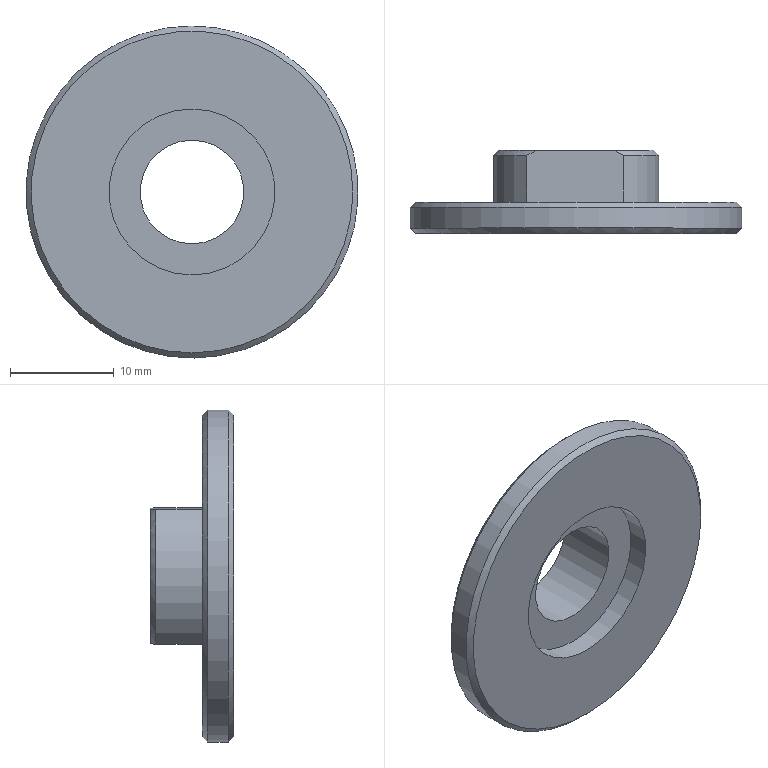Component | NX | LOCK_NUT | 1 solid | 15 faces | box 32 x 8 x 32 mm | volume 2421 mm3 | plane 6 | cylinder 5 | cone 4 | commonest cylinder face diameters 16 x3 32 x1 10 x1
STEP:
#1=CARTESIAN_POINT('',(0.,0.,0.));
#2=DIRECTION('',(0.,0.,1.));
#3=DIRECTION('',(1.,0.,0.));
#4=AXIS2_PLACEMENT_3D('',#1,#2,#3);
#5=CARTESIAN_POINT('',(-431.74,16.4,383.556));
#6=VERTEX_POINT('',#5);
#7=CARTESIAN_POINT('',(-431.676,16.4,378.556));
#8=DIRECTION('',(0.,-1.,0.));
#9=DIRECTION('',(-0.01278,0.,0.9999));
#10=AXIS2_PLACEMENT_3D('',#7,#8,#9);
#11=CIRCLE('',#10,5.);
#12=CARTESIAN_POINT('',(-423.676,16.4,378.658));
#13=DIRECTION('',(0.,-1.,0.));
#14=DIRECTION('',(-0.01278,0.,0.9999));
#15=AXIS2_PLACEMENT_3D('',#12,#13,#14);
#16=PLANE('',#15);
#17=CARTESIAN_POINT('',(-0.,8.));
#18=DIRECTION('',(1.,0.));
#19=AXIS2_PLACEMENT_2D('',#17,#18);
#20=CIRCLE('',#19,5.);
#21=(GEOMETRIC_REPRESENTATION_CONTEXT(2)PARAMETRIC_REPRESENTATION_CONTEXT()REPRESENTATION_CONTEXT('',''));
#22=DEFINITIONAL_REPRESENTATION('',(#20),#21);
#23=PCURVE('',#16,#22);
#24=CARTESIAN_POINT('',(-431.676,16.4,378.556));
#25=DIRECTION('',(0.,-1.,0.));
#26=DIRECTION('',(-0.01278,0.,0.9999));
#27=AXIS2_PLACEMENT_3D('',#24,#25,#26);
#28=CYLINDRICAL_SURFACE('',#27,5.);
#29=CARTESIAN_POINT('',(0.,0.));
#30=DIRECTION('',(1.,0.));
#31=VECTOR('',#30,1.);
#32=LINE('',#29,#31);
#33=(GEOMETRIC_REPRESENTATION_CONTEXT(2)PARAMETRIC_REPRESENTATION_CONTEXT()REPRESENTATION_CONTEXT('',''));
#34=DEFINITIONAL_REPRESENTATION('',(#32),#33);
#35=PCURVE('',#28,#34);
#36=SURFACE_CURVE('',#11,(#23,#35),.PCURVE_S1.);
#37=EDGE_CURVE('',#6,#6,#36,.T.);
#38=ORIENTED_EDGE('',*,*,#37,.T.);
#39=EDGE_LOOP('',(#38));
#40=FACE_BOUND('',#39,.T.);
#41=CARTESIAN_POINT('',(-428.017,16.4,385.103));
#42=VERTEX_POINT('',#41);
#43=CARTESIAN_POINT('',(-435.5,16.4,385.008));
#44=VERTEX_POINT('',#43);
#45=CARTESIAN_POINT('',(-423.759,16.4,385.158));
#46=DIRECTION('',(-0.9999,0.,-0.01278));
#47=VECTOR('',#46,1.);
#48=LINE('',#45,#47);
#49=CARTESIAN_POINT('',(6.5,-0.));
#50=DIRECTION('',(-0.,1.));
#51=VECTOR('',#50,1.);
#52=LINE('',#49,#51);
#53=(GEOMETRIC_REPRESENTATION_CONTEXT(2)PARAMETRIC_REPRESENTATION_CONTEXT()REPRESENTATION_CONTEXT('',''));
#54=DEFINITIONAL_REPRESENTATION('',(#52),#53);
#55=PCURVE('',#16,#54);
#56=CARTESIAN_POINT('',(-424.259,17.9,385.151));
#57=DIRECTION('',(-0.01278,0.,0.9999));
#58=DIRECTION('',(0.9999,0.,0.01278));
#59=AXIS2_PLACEMENT_3D('',#56,#57,#58);
#60=PLANE('',#59);
#61=CARTESIAN_POINT('',(0.5,-1.5));
#62=DIRECTION('',(-1.,0.));
#63=VECTOR('',#62,1.);
#64=LINE('',#61,#63);
#65=(GEOMETRIC_REPRESENTATION_CONTEXT(2)PARAMETRIC_REPRESENTATION_CONTEXT()REPRESENTATION_CONTEXT('',''));
#66=DEFINITIONAL_REPRESENTATION('',(#64),#65);
#67=PCURVE('',#60,#66);
#68=SURFACE_CURVE('',#48,(#55,#67),.PCURVE_S1.);
#69=EDGE_CURVE('',#42,#44,#68,.T.);
#70=ORIENTED_EDGE('',*,*,#69,.F.);
#71=CARTESIAN_POINT('',(-427.851,16.4,372.104));
#72=VERTEX_POINT('',#71);
#73=CARTESIAN_POINT('',(-431.676,16.4,378.556));
#74=DIRECTION('',(0.,1.,0.));
#75=DIRECTION('',(-0.01278,0.,0.9999));
#76=AXIS2_PLACEMENT_3D('',#73,#74,#75);
#77=CIRCLE('',#76,7.5);
#78=CARTESIAN_POINT('',(7.5,8.));
#79=CARTESIAN_POINT('',(7.5,-4.99));
#80=CARTESIAN_POINT('',(-3.75,1.505));
#81=CARTESIAN_POINT('',(-15.,8.));
#82=CARTESIAN_POINT('',(-3.75,14.495));
#83=CARTESIAN_POINT('',(7.5,20.99));
#84=CARTESIAN_POINT('',(7.5,8.));
#85=(BOUNDED_CURVE()B_SPLINE_CURVE(2,(#78,#79,#80,#81,#82,#83,#84),.UNSPECIFIED.,.T.,.F.)B_SPLINE_CURVE_WITH_KNOTS((1,2,2,2,2,1),(-2.094,0.,2.094,4.189,6.283,8.378),.UNSPECIFIED.)CURVE()GEOMETRIC_REPRESENTATION_ITEM()RATIONAL_B_SPLINE_CURVE((1.,0.5,1.,0.5,1.,0.5,1.))REPRESENTATION_ITEM(''));
#86=(GEOMETRIC_REPRESENTATION_CONTEXT(2)PARAMETRIC_REPRESENTATION_CONTEXT()REPRESENTATION_CONTEXT('',''));
#87=DEFINITIONAL_REPRESENTATION('',(#85),#86);
#88=PCURVE('',#16,#87);
#89=CARTESIAN_POINT('',(-431.676,16.4,378.556));
#90=DIRECTION('',(0.,-1.,0.));
#91=DIRECTION('',(-0.01278,0.,0.9999));
#92=AXIS2_PLACEMENT_3D('',#89,#90,#91);
#93=CONICAL_SURFACE('',#92,7.5,0.7854);
#94=CARTESIAN_POINT('',(6.283,-0.));
#95=DIRECTION('',(-1.,0.));
#96=VECTOR('',#95,1.);
#97=LINE('',#94,#96);
#98=(GEOMETRIC_REPRESENTATION_CONTEXT(2)PARAMETRIC_REPRESENTATION_CONTEXT()REPRESENTATION_CONTEXT('',''));
#99=DEFINITIONAL_REPRESENTATION('',(#97),#98);
#100=PCURVE('',#93,#99);
#101=SURFACE_CURVE('',#77,(#88,#100),.PCURVE_S1.);
#102=EDGE_CURVE('',#42,#72,#101,.T.);
#103=ORIENTED_EDGE('',*,*,#102,.T.);
#104=CARTESIAN_POINT('',(-435.334,16.4,372.009));
#105=VERTEX_POINT('',#104);
#106=CARTESIAN_POINT('',(-423.593,16.4,372.159));
#107=DIRECTION('',(0.9999,0.,0.01278));
#108=VECTOR('',#107,1.);
#109=LINE('',#106,#108);
#110=CARTESIAN_POINT('',(-6.5,0.));
#111=DIRECTION('',(-0.,-1.));
#112=VECTOR('',#111,1.);
#113=LINE('',#110,#112);
#114=(GEOMETRIC_REPRESENTATION_CONTEXT(2)PARAMETRIC_REPRESENTATION_CONTEXT()REPRESENTATION_CONTEXT('',''));
#115=DEFINITIONAL_REPRESENTATION('',(#113),#114);
#116=PCURVE('',#16,#115);
#117=CARTESIAN_POINT('',(-440.592,17.9,371.941));
#118=DIRECTION('',(0.01278,0.,-0.9999));
#119=DIRECTION('',(-0.9999,0.,-0.01278));
#120=AXIS2_PLACEMENT_3D('',#117,#118,#119);
#121=PLANE('',#120);
#122=CARTESIAN_POINT('',(-17.,-1.5));
#123=DIRECTION('',(-1.,0.));
#124=VECTOR('',#123,1.);
#125=LINE('',#122,#124);
#126=(GEOMETRIC_REPRESENTATION_CONTEXT(2)PARAMETRIC_REPRESENTATION_CONTEXT()REPRESENTATION_CONTEXT('',''));
#127=DEFINITIONAL_REPRESENTATION('',(#125),#126);
#128=PCURVE('',#121,#127);
#129=SURFACE_CURVE('',#109,(#116,#128),.PCURVE_S1.);
#130=EDGE_CURVE('',#105,#72,#129,.T.);
#131=ORIENTED_EDGE('',*,*,#130,.F.);
#132=CARTESIAN_POINT('',(-431.676,16.4,378.556));
#133=DIRECTION('',(0.,1.,0.));
#134=DIRECTION('',(-0.01278,0.,0.9999));
#135=AXIS2_PLACEMENT_3D('',#132,#133,#134);
#136=CIRCLE('',#135,7.5);
#137=CARTESIAN_POINT('',(7.5,8.));
#138=CARTESIAN_POINT('',(7.5,-4.99));
#139=CARTESIAN_POINT('',(-3.75,1.505));
#140=CARTESIAN_POINT('',(-15.,8.));
#141=CARTESIAN_POINT('',(-3.75,14.495));
#142=CARTESIAN_POINT('',(7.5,20.99));
#143=CARTESIAN_POINT('',(7.5,8.));
#144=(BOUNDED_CURVE()B_SPLINE_CURVE(2,(#137,#138,#139,#140,#141,#142,#143),.UNSPECIFIED.,.T.,.F.)B_SPLINE_CURVE_WITH_KNOTS((1,2,2,2,2,1),(-2.094,0.,2.094,4.189,6.283,8.378),.UNSPECIFIED.)CURVE()GEOMETRIC_REPRESENTATION_ITEM()RATIONAL_B_SPLINE_CURVE((1.,0.5,1.,0.5,1.,0.5,1.))REPRESENTATION_ITEM(''));
#145=(GEOMETRIC_REPRESENTATION_CONTEXT(2)PARAMETRIC_REPRESENTATION_CONTEXT()REPRESENTATION_CONTEXT('',''));
#146=DEFINITIONAL_REPRESENTATION('',(#144),#145);
#147=PCURVE('',#16,#146);
#148=CARTESIAN_POINT('',(-431.676,16.4,378.556));
#149=DIRECTION('',(0.,-1.,0.));
#150=DIRECTION('',(-0.01278,0.,0.9999));
#151=AXIS2_PLACEMENT_3D('',#148,#149,#150);
#152=CONICAL_SURFACE('',#151,7.5,0.7854);
#153=CARTESIAN_POINT('',(6.283,0.));
#154=DIRECTION('',(-1.,-0.));
#155=VECTOR('',#154,1.);
#156=LINE('',#153,#155);
#157=(GEOMETRIC_REPRESENTATION_CONTEXT(2)PARAMETRIC_REPRESENTATION_CONTEXT()REPRESENTATION_CONTEXT('',''));
#158=DEFINITIONAL_REPRESENTATION('',(#156),#157);
#159=PCURVE('',#152,#158);
#160=SURFACE_CURVE('',#136,(#147,#159),.PCURVE_S1.);
#161=EDGE_CURVE('',#105,#44,#160,.T.);
#162=ORIENTED_EDGE('',*,*,#161,.T.);
#163=EDGE_LOOP('',(#70,#103,#131,#162));
#164=FACE_BOUND('',#163,.T.);
#165=ADVANCED_FACE('',(#40,#164),#16,.F.);
#166=CARTESIAN_POINT('',(-426.929,15.9,372.116));
#167=VERTEX_POINT('',#166);
#168=CARTESIAN_POINT('',(-426.929,11.4,372.116));
#169=VERTEX_POINT('',#168);
#170=CARTESIAN_POINT('',(-426.929,8.4,372.116));
#171=DIRECTION('',(0.,-1.,0.));
#172=VECTOR('',#171,1.);
#173=LINE('',#170,#172);
#174=CARTESIAN_POINT('',(-431.676,8.4,378.556));
#175=DIRECTION('',(0.,1.,0.));
#176=DIRECTION('',(0.01278,0.,-0.9999));
#177=AXIS2_PLACEMENT_3D('',#174,#175,#176);
#178=CYLINDRICAL_SURFACE('',#177,8.);
#179=CARTESIAN_POINT('',(5.661,0.));
#180=DIRECTION('',(0.,-1.));
#181=VECTOR('',#180,1.);
#182=LINE('',#179,#181);
#183=(GEOMETRIC_REPRESENTATION_CONTEXT(2)PARAMETRIC_REPRESENTATION_CONTEXT()REPRESENTATION_CONTEXT('',''));
#184=DEFINITIONAL_REPRESENTATION('',(#182),#183);
#185=PCURVE('',#178,#184);
#186=CARTESIAN_POINT('',(-13.664,-9.5));
#187=DIRECTION('',(0.,-1.));
#188=VECTOR('',#187,1.);
#189=LINE('',#186,#188);
#190=(GEOMETRIC_REPRESENTATION_CONTEXT(2)PARAMETRIC_REPRESENTATION_CONTEXT()REPRESENTATION_CONTEXT('',''));
#191=DEFINITIONAL_REPRESENTATION('',(#189),#190);
#192=PCURVE('',#121,#191);
#193=SURFACE_CURVE('',#173,(#185,#192),.PCURVE_S1.);
#194=EDGE_CURVE('',#167,#169,#193,.T.);
#195=ORIENTED_EDGE('',*,*,#194,.F.);
#196=CARTESIAN_POINT('',(-427.095,15.9,385.115));
#197=VERTEX_POINT('',#196);
#198=CARTESIAN_POINT('',(-431.676,15.9,378.556));
#199=DIRECTION('',(0.,-1.,0.));
#200=DIRECTION('',(-0.01278,0.,0.9999));
#201=AXIS2_PLACEMENT_3D('',#198,#199,#200);
#202=CIRCLE('',#201,8.);
#203=CARTESIAN_POINT('',(9.425,7.5));
#204=DIRECTION('',(-1.,0.));
#205=VECTOR('',#204,1.);
#206=LINE('',#203,#205);
#207=(GEOMETRIC_REPRESENTATION_CONTEXT(2)PARAMETRIC_REPRESENTATION_CONTEXT()REPRESENTATION_CONTEXT('',''));
#208=DEFINITIONAL_REPRESENTATION('',(#206),#207);
#209=PCURVE('',#178,#208);
#210=CARTESIAN_POINT('',(-0.,0.5));
#211=DIRECTION('',(1.,-0.));
#212=VECTOR('',#211,1.);
#213=LINE('',#210,#212);
#214=(GEOMETRIC_REPRESENTATION_CONTEXT(2)PARAMETRIC_REPRESENTATION_CONTEXT()REPRESENTATION_CONTEXT('',''));
#215=DEFINITIONAL_REPRESENTATION('',(#213),#214);
#216=PCURVE('',#93,#215);
#217=SURFACE_CURVE('',#202,(#209,#216),.PCURVE_S1.);
#218=EDGE_CURVE('',#167,#197,#217,.T.);
#219=ORIENTED_EDGE('',*,*,#218,.T.);
#220=CARTESIAN_POINT('',(-427.095,11.4,385.115));
#221=VERTEX_POINT('',#220);
#222=CARTESIAN_POINT('',(-427.095,8.4,385.115));
#223=DIRECTION('',(0.,1.,0.));
#224=VECTOR('',#223,1.);
#225=LINE('',#222,#224);
#226=CARTESIAN_POINT('',(3.764,0.));
#227=DIRECTION('',(0.,1.));
#228=VECTOR('',#227,1.);
#229=LINE('',#226,#228);
#230=(GEOMETRIC_REPRESENTATION_CONTEXT(2)PARAMETRIC_REPRESENTATION_CONTEXT()REPRESENTATION_CONTEXT('',''));
#231=DEFINITIONAL_REPRESENTATION('',(#229),#230);
#232=PCURVE('',#178,#231);
#233=CARTESIAN_POINT('',(-2.836,-9.5));
#234=DIRECTION('',(0.,1.));
#235=VECTOR('',#234,1.);
#236=LINE('',#233,#235);
#237=(GEOMETRIC_REPRESENTATION_CONTEXT(2)PARAMETRIC_REPRESENTATION_CONTEXT()REPRESENTATION_CONTEXT('',''));
#238=DEFINITIONAL_REPRESENTATION('',(#236),#237);
#239=PCURVE('',#60,#238);
#240=SURFACE_CURVE('',#225,(#232,#239),.PCURVE_S1.);
#241=EDGE_CURVE('',#221,#197,#240,.T.);
#242=ORIENTED_EDGE('',*,*,#241,.F.);
#243=CARTESIAN_POINT('',(-431.676,11.4,378.556));
#244=DIRECTION('',(0.,1.,0.));
#245=DIRECTION('',(0.01278,0.,-0.9999));
#246=AXIS2_PLACEMENT_3D('',#243,#244,#245);
#247=CIRCLE('',#246,8.);
#248=CARTESIAN_POINT('',(0.,3.));
#249=DIRECTION('',(1.,0.));
#250=VECTOR('',#249,1.);
#251=LINE('',#248,#250);
#252=(GEOMETRIC_REPRESENTATION_CONTEXT(2)PARAMETRIC_REPRESENTATION_CONTEXT()REPRESENTATION_CONTEXT('',''));
#253=DEFINITIONAL_REPRESENTATION('',(#251),#252);
#254=PCURVE('',#178,#253);
#255=CARTESIAN_POINT('',(-415.677,11.4,378.76));
#256=DIRECTION('',(0.,-1.,0.));
#257=DIRECTION('',(-0.01278,0.,0.9999));
#258=AXIS2_PLACEMENT_3D('',#255,#256,#257);
#259=PLANE('',#258);
#260=CARTESIAN_POINT('',(-8.,16.));
#261=CARTESIAN_POINT('',(-8.,29.856));
#262=CARTESIAN_POINT('',(4.,22.928));
#263=CARTESIAN_POINT('',(16.,16.));
#264=CARTESIAN_POINT('',(4.,9.072));
#265=CARTESIAN_POINT('',(-8.,2.144));
#266=CARTESIAN_POINT('',(-8.,16.));
#267=(BOUNDED_CURVE()B_SPLINE_CURVE(2,(#260,#261,#262,#263,#264,#265,#266),.UNSPECIFIED.,.T.,.F.)B_SPLINE_CURVE_WITH_KNOTS((1,2,2,2,2,1),(-2.094,0.,2.094,4.189,6.283,8.378),.UNSPECIFIED.)CURVE()GEOMETRIC_REPRESENTATION_ITEM()RATIONAL_B_SPLINE_CURVE((1.,0.5,1.,0.5,1.,0.5,1.))REPRESENTATION_ITEM(''));
#268=(GEOMETRIC_REPRESENTATION_CONTEXT(2)PARAMETRIC_REPRESENTATION_CONTEXT()REPRESENTATION_CONTEXT('',''));
#269=DEFINITIONAL_REPRESENTATION('',(#267),#268);
#270=PCURVE('',#259,#269);
#271=SURFACE_CURVE('',#247,(#254,#270),.PCURVE_S1.);
#272=EDGE_CURVE('',#221,#169,#271,.T.);
#273=ORIENTED_EDGE('',*,*,#272,.T.);
#274=EDGE_LOOP('',(#195,#219,#242,#273));
#275=FACE_BOUND('',#274,.T.);
#276=ADVANCED_FACE('',(#275),#178,.T.);
#277=CARTESIAN_POINT('',(-436.422,15.9,384.996));
#278=VERTEX_POINT('',#277);
#279=CARTESIAN_POINT('',(-436.422,11.4,384.996));
#280=VERTEX_POINT('',#279);
#281=CARTESIAN_POINT('',(-436.422,8.4,384.996));
#282=DIRECTION('',(0.,-1.,0.));
#283=VECTOR('',#282,1.);
#284=LINE('',#281,#283);
#285=CARTESIAN_POINT('',(-431.676,8.4,378.556));
#286=DIRECTION('',(0.,1.,0.));
#287=DIRECTION('',(0.01278,0.,-0.9999));
#288=AXIS2_PLACEMENT_3D('',#285,#286,#287);
#289=CYLINDRICAL_SURFACE('',#288,8.);
#290=CARTESIAN_POINT('',(2.519,0.));
#291=DIRECTION('',(0.,-1.));
#292=VECTOR('',#291,1.);
#293=LINE('',#290,#292);
#294=(GEOMETRIC_REPRESENTATION_CONTEXT(2)PARAMETRIC_REPRESENTATION_CONTEXT()REPRESENTATION_CONTEXT('',''));
#295=DEFINITIONAL_REPRESENTATION('',(#293),#294);
#296=PCURVE('',#289,#295);
#297=CARTESIAN_POINT('',(-12.164,-9.5));
#298=DIRECTION('',(0.,-1.));
#299=VECTOR('',#298,1.);
#300=LINE('',#297,#299);
#301=(GEOMETRIC_REPRESENTATION_CONTEXT(2)PARAMETRIC_REPRESENTATION_CONTEXT()REPRESENTATION_CONTEXT('',''));
#302=DEFINITIONAL_REPRESENTATION('',(#300),#301);
#303=PCURVE('',#60,#302);
#304=SURFACE_CURVE('',#284,(#296,#303),.PCURVE_S1.);
#305=EDGE_CURVE('',#278,#280,#304,.T.);
#306=ORIENTED_EDGE('',*,*,#305,.F.);
#307=CARTESIAN_POINT('',(-436.256,15.9,371.997));
#308=VERTEX_POINT('',#307);
#309=CARTESIAN_POINT('',(-431.676,15.9,378.556));
#310=DIRECTION('',(0.,-1.,0.));
#311=DIRECTION('',(-0.01278,0.,0.9999));
#312=AXIS2_PLACEMENT_3D('',#309,#310,#311);
#313=CIRCLE('',#312,8.);
#314=CARTESIAN_POINT('',(3.142,7.5));
#315=DIRECTION('',(-1.,0.));
#316=VECTOR('',#315,1.);
#317=LINE('',#314,#316);
#318=(GEOMETRIC_REPRESENTATION_CONTEXT(2)PARAMETRIC_REPRESENTATION_CONTEXT()REPRESENTATION_CONTEXT('',''));
#319=DEFINITIONAL_REPRESENTATION('',(#317),#318);
#320=PCURVE('',#289,#319);
#321=CARTESIAN_POINT('',(-0.,0.5));
#322=DIRECTION('',(1.,0.));
#323=VECTOR('',#322,1.);
#324=LINE('',#321,#323);
#325=(GEOMETRIC_REPRESENTATION_CONTEXT(2)PARAMETRIC_REPRESENTATION_CONTEXT()REPRESENTATION_CONTEXT('',''));
#326=DEFINITIONAL_REPRESENTATION('',(#324),#325);
#327=PCURVE('',#152,#326);
#328=SURFACE_CURVE('',#313,(#320,#327),.PCURVE_S1.);
#329=EDGE_CURVE('',#278,#308,#328,.T.);
#330=ORIENTED_EDGE('',*,*,#329,.T.);
#331=CARTESIAN_POINT('',(-436.256,11.4,371.997));
#332=VERTEX_POINT('',#331);
#333=CARTESIAN_POINT('',(-436.256,8.4,371.997));
#334=DIRECTION('',(0.,1.,0.));
#335=VECTOR('',#334,1.);
#336=LINE('',#333,#335);
#337=CARTESIAN_POINT('',(0.6224,0.));
#338=DIRECTION('',(0.,1.));
#339=VECTOR('',#338,1.);
#340=LINE('',#337,#339);
#341=(GEOMETRIC_REPRESENTATION_CONTEXT(2)PARAMETRIC_REPRESENTATION_CONTEXT()REPRESENTATION_CONTEXT('',''));
#342=DEFINITIONAL_REPRESENTATION('',(#340),#341);
#343=PCURVE('',#289,#342);
#344=CARTESIAN_POINT('',(-4.336,-9.5));
#345=DIRECTION('',(0.,1.));
#346=VECTOR('',#345,1.);
#347=LINE('',#344,#346);
#348=(GEOMETRIC_REPRESENTATION_CONTEXT(2)PARAMETRIC_REPRESENTATION_CONTEXT()REPRESENTATION_CONTEXT('',''));
#349=DEFINITIONAL_REPRESENTATION('',(#347),#348);
#350=PCURVE('',#121,#349);
#351=SURFACE_CURVE('',#336,(#343,#350),.PCURVE_S1.);
#352=EDGE_CURVE('',#332,#308,#351,.T.);
#353=ORIENTED_EDGE('',*,*,#352,.F.);
#354=CARTESIAN_POINT('',(-431.676,11.4,378.556));
#355=DIRECTION('',(0.,1.,0.));
#356=DIRECTION('',(0.01278,0.,-0.9999));
#357=AXIS2_PLACEMENT_3D('',#354,#355,#356);
#358=CIRCLE('',#357,8.);
#359=CARTESIAN_POINT('',(-0.,3.));
#360=DIRECTION('',(1.,0.));
#361=VECTOR('',#360,1.);
#362=LINE('',#359,#361);
#363=(GEOMETRIC_REPRESENTATION_CONTEXT(2)PARAMETRIC_REPRESENTATION_CONTEXT()REPRESENTATION_CONTEXT('',''));
#364=DEFINITIONAL_REPRESENTATION('',(#362),#363);
#365=PCURVE('',#289,#364);
#366=CARTESIAN_POINT('',(-8.,16.));
#367=CARTESIAN_POINT('',(-8.,29.856));
#368=CARTESIAN_POINT('',(4.,22.928));
#369=CARTESIAN_POINT('',(16.,16.));
#370=CARTESIAN_POINT('',(4.,9.072));
#371=CARTESIAN_POINT('',(-8.,2.144));
#372=CARTESIAN_POINT('',(-8.,16.));
#373=(BOUNDED_CURVE()B_SPLINE_CURVE(2,(#366,#367,#368,#369,#370,#371,#372),.UNSPECIFIED.,.T.,.F.)B_SPLINE_CURVE_WITH_KNOTS((1,2,2,2,2,1),(-2.094,0.,2.094,4.189,6.283,8.378),.UNSPECIFIED.)CURVE()GEOMETRIC_REPRESENTATION_ITEM()RATIONAL_B_SPLINE_CURVE((1.,0.5,1.,0.5,1.,0.5,1.))REPRESENTATION_ITEM(''));
#374=(GEOMETRIC_REPRESENTATION_CONTEXT(2)PARAMETRIC_REPRESENTATION_CONTEXT()REPRESENTATION_CONTEXT('',''));
#375=DEFINITIONAL_REPRESENTATION('',(#373),#374);
#376=PCURVE('',#259,#375);
#377=SURFACE_CURVE('',#358,(#365,#376),.PCURVE_S1.);
#378=EDGE_CURVE('',#332,#280,#377,.T.);
#379=ORIENTED_EDGE('',*,*,#378,.T.);
#380=EDGE_LOOP('',(#306,#330,#353,#379));
#381=FACE_BOUND('',#380,.T.);
#382=ADVANCED_FACE('',(#381),#289,.T.);
#383=CARTESIAN_POINT('',(-431.874,11.4,394.055));
#384=VERTEX_POINT('',#383);
#385=CARTESIAN_POINT('',(-431.676,11.4,378.556));
#386=DIRECTION('',(0.,1.,0.));
#387=DIRECTION('',(-0.01278,0.,0.9999));
#388=AXIS2_PLACEMENT_3D('',#385,#386,#387);
#389=CIRCLE('',#388,15.5);
#390=CARTESIAN_POINT('',(15.5,16.));
#391=CARTESIAN_POINT('',(15.5,-10.847));
#392=CARTESIAN_POINT('',(-7.75,2.577));
#393=CARTESIAN_POINT('',(-31.,16.));
#394=CARTESIAN_POINT('',(-7.75,29.423));
#395=CARTESIAN_POINT('',(15.5,42.847));
#396=CARTESIAN_POINT('',(15.5,16.));
#397=(BOUNDED_CURVE()B_SPLINE_CURVE(2,(#390,#391,#392,#393,#394,#395,#396),.UNSPECIFIED.,.T.,.F.)B_SPLINE_CURVE_WITH_KNOTS((1,2,2,2,2,1),(-2.094,0.,2.094,4.189,6.283,8.378),.UNSPECIFIED.)CURVE()GEOMETRIC_REPRESENTATION_ITEM()RATIONAL_B_SPLINE_CURVE((1.,0.5,1.,0.5,1.,0.5,1.))REPRESENTATION_ITEM(''));
#398=(GEOMETRIC_REPRESENTATION_CONTEXT(2)PARAMETRIC_REPRESENTATION_CONTEXT()REPRESENTATION_CONTEXT('',''));
#399=DEFINITIONAL_REPRESENTATION('',(#397),#398);
#400=PCURVE('',#259,#399);
#401=CARTESIAN_POINT('',(-431.676,11.4,378.556));
#402=DIRECTION('',(0.,-1.,0.));
#403=DIRECTION('',(-0.01278,0.,0.9999));
#404=AXIS2_PLACEMENT_3D('',#401,#402,#403);
#405=CONICAL_SURFACE('',#404,15.5,0.7854);
#406=CARTESIAN_POINT('',(6.283,-0.));
#407=DIRECTION('',(-1.,0.));
#408=VECTOR('',#407,1.);
#409=LINE('',#406,#408);
#410=(GEOMETRIC_REPRESENTATION_CONTEXT(2)PARAMETRIC_REPRESENTATION_CONTEXT()REPRESENTATION_CONTEXT('',''));
#411=DEFINITIONAL_REPRESENTATION('',(#409),#410);
#412=PCURVE('',#405,#411);
#413=SURFACE_CURVE('',#389,(#400,#412),.PCURVE_S1.);
#414=EDGE_CURVE('',#384,#384,#413,.T.);
#415=ORIENTED_EDGE('',*,*,#414,.T.);
#416=EDGE_LOOP('',(#415));
#417=FACE_BOUND('',#416,.T.);
#418=ORIENTED_EDGE('',*,*,#272,.F.);
#419=CARTESIAN_POINT('',(-424.259,11.4,385.151));
#420=DIRECTION('',(-0.9999,0.,-0.01278));
#421=VECTOR('',#420,1.);
#422=LINE('',#419,#421);
#423=CARTESIAN_POINT('',(6.5,8.5));
#424=DIRECTION('',(-0.,1.));
#425=VECTOR('',#424,1.);
#426=LINE('',#423,#425);
#427=(GEOMETRIC_REPRESENTATION_CONTEXT(2)PARAMETRIC_REPRESENTATION_CONTEXT()REPRESENTATION_CONTEXT('',''));
#428=DEFINITIONAL_REPRESENTATION('',(#426),#427);
#429=PCURVE('',#259,#428);
#430=CARTESIAN_POINT('',(0.,-6.5));
#431=DIRECTION('',(-1.,0.));
#432=VECTOR('',#431,1.);
#433=LINE('',#430,#432);
#434=(GEOMETRIC_REPRESENTATION_CONTEXT(2)PARAMETRIC_REPRESENTATION_CONTEXT()REPRESENTATION_CONTEXT('',''));
#435=DEFINITIONAL_REPRESENTATION('',(#433),#434);
#436=PCURVE('',#60,#435);
#437=SURFACE_CURVE('',#422,(#429,#436),.PCURVE_S1.);
#438=EDGE_CURVE('',#221,#280,#437,.T.);
#439=ORIENTED_EDGE('',*,*,#438,.T.);
#440=ORIENTED_EDGE('',*,*,#378,.F.);
#441=CARTESIAN_POINT('',(-440.592,11.4,371.941));
#442=DIRECTION('',(0.9999,0.,0.01278));
#443=VECTOR('',#442,1.);
#444=LINE('',#441,#443);
#445=CARTESIAN_POINT('',(-6.5,25.));
#446=DIRECTION('',(-0.,-1.));
#447=VECTOR('',#446,1.);
#448=LINE('',#445,#447);
#449=(GEOMETRIC_REPRESENTATION_CONTEXT(2)PARAMETRIC_REPRESENTATION_CONTEXT()REPRESENTATION_CONTEXT('',''));
#450=DEFINITIONAL_REPRESENTATION('',(#448),#449);
#451=PCURVE('',#259,#450);
#452=CARTESIAN_POINT('',(0.,-6.5));
#453=DIRECTION('',(-1.,0.));
#454=VECTOR('',#453,1.);
#455=LINE('',#452,#454);
#456=(GEOMETRIC_REPRESENTATION_CONTEXT(2)PARAMETRIC_REPRESENTATION_CONTEXT()REPRESENTATION_CONTEXT('',''));
#457=DEFINITIONAL_REPRESENTATION('',(#455),#456);
#458=PCURVE('',#121,#457);
#459=SURFACE_CURVE('',#444,(#451,#458),.PCURVE_S1.);
#460=EDGE_CURVE('',#332,#169,#459,.T.);
#461=ORIENTED_EDGE('',*,*,#460,.T.);
#462=EDGE_LOOP('',(#418,#439,#440,#461));
#463=FACE_BOUND('',#462,.T.);
#464=ADVANCED_FACE('',(#417,#463),#259,.F.);
#465=CARTESIAN_POINT('',(-431.471,8.9,362.557));
#466=VERTEX_POINT('',#465);
#467=CARTESIAN_POINT('',(-431.676,8.9,378.556));
#468=DIRECTION('',(0.,1.,0.));
#469=DIRECTION('',(0.01278,0.,-0.9999));
#470=AXIS2_PLACEMENT_3D('',#467,#468,#469);
#471=CIRCLE('',#470,16.);
#472=CARTESIAN_POINT('',(-431.676,8.4,378.556));
#473=DIRECTION('',(0.,1.,0.));
#474=DIRECTION('',(0.01278,0.,-0.9999));
#475=AXIS2_PLACEMENT_3D('',#472,#473,#474);
#476=CYLINDRICAL_SURFACE('',#475,16.);
#477=CARTESIAN_POINT('',(0.,0.5));
#478=DIRECTION('',(1.,0.));
#479=VECTOR('',#478,1.);
#480=LINE('',#477,#479);
#481=(GEOMETRIC_REPRESENTATION_CONTEXT(2)PARAMETRIC_REPRESENTATION_CONTEXT()REPRESENTATION_CONTEXT('',''));
#482=DEFINITIONAL_REPRESENTATION('',(#480),#481);
#483=PCURVE('',#476,#482);
#484=CARTESIAN_POINT('',(-431.676,8.9,378.556));
#485=DIRECTION('',(0.,1.,0.));
#486=DIRECTION('',(0.01278,0.,-0.9999));
#487=AXIS2_PLACEMENT_3D('',#484,#485,#486);
#488=CONICAL_SURFACE('',#487,16.,0.7854);
#489=CARTESIAN_POINT('',(0.,0.));
#490=DIRECTION('',(1.,0.));
#491=VECTOR('',#490,1.);
#492=LINE('',#489,#491);
#493=(GEOMETRIC_REPRESENTATION_CONTEXT(2)PARAMETRIC_REPRESENTATION_CONTEXT()REPRESENTATION_CONTEXT('',''));
#494=DEFINITIONAL_REPRESENTATION('',(#492),#493);
#495=PCURVE('',#488,#494);
#496=SURFACE_CURVE('',#471,(#483,#495),.PCURVE_S1.);
#497=EDGE_CURVE('',#466,#466,#496,.T.);
#498=ORIENTED_EDGE('',*,*,#497,.T.);
#499=CARTESIAN_POINT('',(-431.471,10.9,362.557));
#500=VERTEX_POINT('',#499);
#501=CARTESIAN_POINT('',(-431.471,8.9,362.557));
#502=CARTESIAN_POINT('',(-431.471,10.9,362.557));
#503=B_SPLINE_CURVE_WITH_KNOTS('',1,(#501,#502),.UNSPECIFIED.,.F.,.F.,(2,2),(0.5,2.5),.PIECEWISE_BEZIER_KNOTS.);
#504=CARTESIAN_POINT('',(6.283,0.));
#505=DIRECTION('',(0.,1.));
#506=VECTOR('',#505,1.);
#507=LINE('',#504,#506);
#508=(GEOMETRIC_REPRESENTATION_CONTEXT(2)PARAMETRIC_REPRESENTATION_CONTEXT()REPRESENTATION_CONTEXT('',''));
#509=DEFINITIONAL_REPRESENTATION('',(#507),#508);
#510=PCURVE('',#476,#509);
#511=CARTESIAN_POINT('',(0.,0.));
#512=DIRECTION('',(0.,1.));
#513=VECTOR('',#512,1.);
#514=LINE('',#511,#513);
#515=(GEOMETRIC_REPRESENTATION_CONTEXT(2)PARAMETRIC_REPRESENTATION_CONTEXT()REPRESENTATION_CONTEXT('',''));
#516=DEFINITIONAL_REPRESENTATION('',(#514),#515);
#517=PCURVE('',#476,#516);
#518=SEAM_CURVE('',#503,(#510,#517),.PCURVE_S1.);
#519=EDGE_CURVE('',#466,#500,#518,.T.);
#520=ORIENTED_EDGE('',*,*,#519,.T.);
#521=CARTESIAN_POINT('',(-431.88,10.9,394.555));
#522=VERTEX_POINT('',#521);
#523=CARTESIAN_POINT('',(-431.676,10.9,378.556));
#524=DIRECTION('',(0.,-1.,0.));
#525=DIRECTION('',(-0.01278,0.,0.9999));
#526=AXIS2_PLACEMENT_3D('',#523,#524,#525);
#527=CIRCLE('',#526,16.);
#528=CARTESIAN_POINT('',(9.425,2.5));
#529=DIRECTION('',(-1.,0.));
#530=VECTOR('',#529,1.);
#531=LINE('',#528,#530);
#532=(GEOMETRIC_REPRESENTATION_CONTEXT(2)PARAMETRIC_REPRESENTATION_CONTEXT()REPRESENTATION_CONTEXT('',''));
#533=DEFINITIONAL_REPRESENTATION('',(#531),#532);
#534=PCURVE('',#476,#533);
#535=CARTESIAN_POINT('',(0.,0.5));
#536=DIRECTION('',(1.,-0.));
#537=VECTOR('',#536,1.);
#538=LINE('',#535,#537);
#539=(GEOMETRIC_REPRESENTATION_CONTEXT(2)PARAMETRIC_REPRESENTATION_CONTEXT()REPRESENTATION_CONTEXT('',''));
#540=DEFINITIONAL_REPRESENTATION('',(#538),#539);
#541=PCURVE('',#405,#540);
#542=SURFACE_CURVE('',#527,(#534,#541),.PCURVE_S1.);
#543=EDGE_CURVE('',#500,#522,#542,.T.);
#544=ORIENTED_EDGE('',*,*,#543,.T.);
#545=CARTESIAN_POINT('',(-431.676,10.9,378.556));
#546=DIRECTION('',(0.,-1.,0.));
#547=DIRECTION('',(-0.01278,0.,0.9999));
#548=AXIS2_PLACEMENT_3D('',#545,#546,#547);
#549=CIRCLE('',#548,16.);
#550=CARTESIAN_POINT('',(3.142,2.5));
#551=DIRECTION('',(-1.,0.));
#552=VECTOR('',#551,1.);
#553=LINE('',#550,#552);
#554=(GEOMETRIC_REPRESENTATION_CONTEXT(2)PARAMETRIC_REPRESENTATION_CONTEXT()REPRESENTATION_CONTEXT('',''));
#555=DEFINITIONAL_REPRESENTATION('',(#553),#554);
#556=PCURVE('',#476,#555);
#557=CARTESIAN_POINT('',(0.,0.5));
#558=DIRECTION('',(1.,0.));
#559=VECTOR('',#558,1.);
#560=LINE('',#557,#559);
#561=(GEOMETRIC_REPRESENTATION_CONTEXT(2)PARAMETRIC_REPRESENTATION_CONTEXT()REPRESENTATION_CONTEXT('',''));
#562=DEFINITIONAL_REPRESENTATION('',(#560),#561);
#563=PCURVE('',#405,#562);
#564=SURFACE_CURVE('',#549,(#556,#563),.PCURVE_S1.);
#565=EDGE_CURVE('',#522,#500,#564,.T.);
#566=ORIENTED_EDGE('',*,*,#565,.T.);
#567=ORIENTED_EDGE('',*,*,#519,.F.);
#568=EDGE_LOOP('',(#498,#520,#544,#566,#567));
#569=FACE_BOUND('',#568,.T.);
#570=ADVANCED_FACE('',(#569),#476,.T.);
#571=CARTESIAN_POINT('',(-431.478,8.4,363.057));
#572=VERTEX_POINT('',#571);
#573=CARTESIAN_POINT('',(-431.676,8.4,378.556));
#574=DIRECTION('',(0.,-1.,0.));
#575=DIRECTION('',(0.01278,0.,-0.9999));
#576=AXIS2_PLACEMENT_3D('',#573,#574,#575);
#577=CIRCLE('',#576,15.5);
#578=CARTESIAN_POINT('',(-423.676,8.4,378.658));
#579=DIRECTION('',(0.,1.,0.));
#580=DIRECTION('',(0.01278,0.,-0.9999));
#581=AXIS2_PLACEMENT_3D('',#578,#579,#580);
#582=PLANE('',#581);
#583=CARTESIAN_POINT('',(15.5,8.));
#584=CARTESIAN_POINT('',(15.5,-18.847));
#585=CARTESIAN_POINT('',(-7.75,-5.423));
#586=CARTESIAN_POINT('',(-31.,8.));
#587=CARTESIAN_POINT('',(-7.75,21.423));
#588=CARTESIAN_POINT('',(15.5,34.847));
#589=CARTESIAN_POINT('',(15.5,8.));
#590=(BOUNDED_CURVE()B_SPLINE_CURVE(2,(#583,#584,#585,#586,#587,#588,#589),.UNSPECIFIED.,.T.,.F.)B_SPLINE_CURVE_WITH_KNOTS((1,2,2,2,2,1),(-2.094,0.,2.094,4.189,6.283,8.378),.UNSPECIFIED.)CURVE()GEOMETRIC_REPRESENTATION_ITEM()RATIONAL_B_SPLINE_CURVE((1.,0.5,1.,0.5,1.,0.5,1.))REPRESENTATION_ITEM(''));
#591=(GEOMETRIC_REPRESENTATION_CONTEXT(2)PARAMETRIC_REPRESENTATION_CONTEXT()REPRESENTATION_CONTEXT('',''));
#592=DEFINITIONAL_REPRESENTATION('',(#590),#591);
#593=PCURVE('',#582,#592);
#594=CARTESIAN_POINT('',(6.283,-0.5));
#595=DIRECTION('',(-1.,0.));
#596=VECTOR('',#595,1.);
#597=LINE('',#594,#596);
#598=(GEOMETRIC_REPRESENTATION_CONTEXT(2)PARAMETRIC_REPRESENTATION_CONTEXT()REPRESENTATION_CONTEXT('',''));
#599=DEFINITIONAL_REPRESENTATION('',(#597),#598);
#600=PCURVE('',#488,#599);
#601=SURFACE_CURVE('',#577,(#593,#600),.PCURVE_S1.);
#602=EDGE_CURVE('',#572,#572,#601,.T.);
#603=ORIENTED_EDGE('',*,*,#602,.T.);
#604=EDGE_LOOP('',(#603));
#605=FACE_BOUND('',#604,.T.);
#606=CARTESIAN_POINT('',(-431.573,8.4,370.557));
#607=VERTEX_POINT('',#606);
#608=CARTESIAN_POINT('',(-431.676,8.4,378.556));
#609=DIRECTION('',(0.,1.,0.));
#610=DIRECTION('',(0.01278,0.,-0.9999));
#611=AXIS2_PLACEMENT_3D('',#608,#609,#610);
#612=CIRCLE('',#611,8.);
#613=CARTESIAN_POINT('',(0.,8.));
#614=DIRECTION('',(1.,-0.));
#615=AXIS2_PLACEMENT_2D('',#613,#614);
#616=CIRCLE('',#615,8.);
#617=(GEOMETRIC_REPRESENTATION_CONTEXT(2)PARAMETRIC_REPRESENTATION_CONTEXT()REPRESENTATION_CONTEXT('',''));
#618=DEFINITIONAL_REPRESENTATION('',(#616),#617);
#619=PCURVE('',#582,#618);
#620=CARTESIAN_POINT('',(-431.676,8.4,378.556));
#621=DIRECTION('',(0.,1.,0.));
#622=DIRECTION('',(0.01278,0.,-0.9999));
#623=AXIS2_PLACEMENT_3D('',#620,#621,#622);
#624=CYLINDRICAL_SURFACE('',#623,8.);
#625=CARTESIAN_POINT('',(0.,0.));
#626=DIRECTION('',(1.,0.));
#627=VECTOR('',#626,1.);
#628=LINE('',#625,#627);
#629=(GEOMETRIC_REPRESENTATION_CONTEXT(2)PARAMETRIC_REPRESENTATION_CONTEXT()REPRESENTATION_CONTEXT('',''));
#630=DEFINITIONAL_REPRESENTATION('',(#628),#629);
#631=PCURVE('',#624,#630);
#632=SURFACE_CURVE('',#612,(#619,#631),.PCURVE_S1.);
#633=EDGE_CURVE('',#607,#607,#632,.T.);
#634=ORIENTED_EDGE('',*,*,#633,.T.);
#635=EDGE_LOOP('',(#634));
#636=FACE_BOUND('',#635,.T.);
#637=ADVANCED_FACE('',(#605,#636),#582,.F.);
#638=ORIENTED_EDGE('',*,*,#633,.T.);
#639=CARTESIAN_POINT('',(-431.573,10.4,370.557));
#640=VERTEX_POINT('',#639);
#641=CARTESIAN_POINT('',(-431.573,8.4,370.557));
#642=CARTESIAN_POINT('',(-431.573,10.4,370.557));
#643=B_SPLINE_CURVE_WITH_KNOTS('',1,(#641,#642),.UNSPECIFIED.,.F.,.F.,(2,2),(0.,2.),.PIECEWISE_BEZIER_KNOTS.);
#644=CARTESIAN_POINT('',(6.283,0.));
#645=DIRECTION('',(0.,1.));
#646=VECTOR('',#645,1.);
#647=LINE('',#644,#646);
#648=(GEOMETRIC_REPRESENTATION_CONTEXT(2)PARAMETRIC_REPRESENTATION_CONTEXT()REPRESENTATION_CONTEXT('',''));
#649=DEFINITIONAL_REPRESENTATION('',(#647),#648);
#650=PCURVE('',#624,#649);
#651=CARTESIAN_POINT('',(0.,0.));
#652=DIRECTION('',(0.,1.));
#653=VECTOR('',#652,1.);
#654=LINE('',#651,#653);
#655=(GEOMETRIC_REPRESENTATION_CONTEXT(2)PARAMETRIC_REPRESENTATION_CONTEXT()REPRESENTATION_CONTEXT('',''));
#656=DEFINITIONAL_REPRESENTATION('',(#654),#655);
#657=PCURVE('',#624,#656);
#658=SEAM_CURVE('',#643,(#650,#657),.PCURVE_S1.);
#659=EDGE_CURVE('',#607,#640,#658,.T.);
#660=ORIENTED_EDGE('',*,*,#659,.T.);
#661=CARTESIAN_POINT('',(-431.676,10.4,378.556));
#662=DIRECTION('',(0.,1.,0.));
#663=DIRECTION('',(0.01278,0.,-0.9999));
#664=AXIS2_PLACEMENT_3D('',#661,#662,#663);
#665=CIRCLE('',#664,8.);
#666=CARTESIAN_POINT('',(0.,2.));
#667=DIRECTION('',(1.,0.));
#668=VECTOR('',#667,1.);
#669=LINE('',#666,#668);
#670=(GEOMETRIC_REPRESENTATION_CONTEXT(2)PARAMETRIC_REPRESENTATION_CONTEXT()REPRESENTATION_CONTEXT('',''));
#671=DEFINITIONAL_REPRESENTATION('',(#669),#670);
#672=PCURVE('',#624,#671);
#673=CARTESIAN_POINT('',(-431.676,10.4,378.556));
#674=DIRECTION('',(0.,1.,0.));
#675=DIRECTION('',(0.01278,0.,-0.9999));
#676=AXIS2_PLACEMENT_3D('',#673,#674,#675);
#677=PLANE('',#676);
#678=CARTESIAN_POINT('',(0.,0.));
#679=DIRECTION('',(1.,-0.));
#680=AXIS2_PLACEMENT_2D('',#678,#679);
#681=CIRCLE('',#680,8.);
#682=(GEOMETRIC_REPRESENTATION_CONTEXT(2)PARAMETRIC_REPRESENTATION_CONTEXT()REPRESENTATION_CONTEXT('',''));
#683=DEFINITIONAL_REPRESENTATION('',(#681),#682);
#684=PCURVE('',#677,#683);
#685=SURFACE_CURVE('',#665,(#672,#684),.PCURVE_S1.);
#686=EDGE_CURVE('',#640,#640,#685,.T.);
#687=ORIENTED_EDGE('',*,*,#686,.F.);
#688=ORIENTED_EDGE('',*,*,#659,.F.);
#689=EDGE_LOOP('',(#638,#660,#687,#688));
#690=FACE_BOUND('',#689,.F.);
#691=ADVANCED_FACE('',(#690),#624,.F.);
#692=CARTESIAN_POINT('',(-431.612,10.4,373.556));
#693=VERTEX_POINT('',#692);
#694=CARTESIAN_POINT('',(-431.74,10.4,383.556));
#695=VERTEX_POINT('',#694);
#696=CARTESIAN_POINT('',(-431.676,10.4,378.556));
#697=DIRECTION('',(0.,1.,0.));
#698=DIRECTION('',(0.01278,0.,-0.9999));
#699=AXIS2_PLACEMENT_3D('',#696,#697,#698);
#700=CIRCLE('',#699,5.);
#701=CARTESIAN_POINT('',(0.,0.));
#702=DIRECTION('',(1.,-0.));
#703=AXIS2_PLACEMENT_2D('',#701,#702);
#704=CIRCLE('',#703,5.);
#705=(GEOMETRIC_REPRESENTATION_CONTEXT(2)PARAMETRIC_REPRESENTATION_CONTEXT()REPRESENTATION_CONTEXT('',''));
#706=DEFINITIONAL_REPRESENTATION('',(#704),#705);
#707=PCURVE('',#677,#706);
#708=CARTESIAN_POINT('',(3.142,6.));
#709=DIRECTION('',(-1.,0.));
#710=VECTOR('',#709,1.);
#711=LINE('',#708,#710);
#712=(GEOMETRIC_REPRESENTATION_CONTEXT(2)PARAMETRIC_REPRESENTATION_CONTEXT()REPRESENTATION_CONTEXT('',''));
#713=DEFINITIONAL_REPRESENTATION('',(#711),#712);
#714=PCURVE('',#28,#713);
#715=SURFACE_CURVE('',#700,(#707,#714),.PCURVE_S1.);
#716=EDGE_CURVE('',#693,#695,#715,.T.);
#717=ORIENTED_EDGE('',*,*,#716,.T.);
#718=CARTESIAN_POINT('',(-431.676,10.4,378.556));
#719=DIRECTION('',(0.,1.,0.));
#720=DIRECTION('',(0.01278,0.,-0.9999));
#721=AXIS2_PLACEMENT_3D('',#718,#719,#720);
#722=CIRCLE('',#721,5.);
#723=CARTESIAN_POINT('',(0.,0.));
#724=DIRECTION('',(1.,-0.));
#725=AXIS2_PLACEMENT_2D('',#723,#724);
#726=CIRCLE('',#725,5.);
#727=(GEOMETRIC_REPRESENTATION_CONTEXT(2)PARAMETRIC_REPRESENTATION_CONTEXT()REPRESENTATION_CONTEXT('',''));
#728=DEFINITIONAL_REPRESENTATION('',(#726),#727);
#729=PCURVE('',#677,#728);
#730=CARTESIAN_POINT('',(9.425,6.));
#731=DIRECTION('',(-1.,0.));
#732=VECTOR('',#731,1.);
#733=LINE('',#730,#732);
#734=(GEOMETRIC_REPRESENTATION_CONTEXT(2)PARAMETRIC_REPRESENTATION_CONTEXT()REPRESENTATION_CONTEXT('',''));
#735=DEFINITIONAL_REPRESENTATION('',(#733),#734);
#736=PCURVE('',#28,#735);
#737=SURFACE_CURVE('',#722,(#729,#736),.PCURVE_S1.);
#738=EDGE_CURVE('',#695,#693,#737,.T.);
#739=ORIENTED_EDGE('',*,*,#738,.T.);
#740=EDGE_LOOP('',(#717,#739));
#741=FACE_BOUND('',#740,.T.);
#742=ORIENTED_EDGE('',*,*,#686,.F.);
#743=EDGE_LOOP('',(#742));
#744=FACE_BOUND('',#743,.T.);
#745=ADVANCED_FACE('',(#741,#744),#677,.F.);
#746=ORIENTED_EDGE('',*,*,#37,.T.);
#747=CARTESIAN_POINT('',(-431.74,16.4,383.556));
#748=CARTESIAN_POINT('',(-431.74,10.4,383.556));
#749=B_SPLINE_CURVE_WITH_KNOTS('',1,(#747,#748),.UNSPECIFIED.,.F.,.F.,(2,2),(0.,6.),.PIECEWISE_BEZIER_KNOTS.);
#750=CARTESIAN_POINT('',(6.283,0.));
#751=DIRECTION('',(0.,1.));
#752=VECTOR('',#751,1.);
#753=LINE('',#750,#752);
#754=(GEOMETRIC_REPRESENTATION_CONTEXT(2)PARAMETRIC_REPRESENTATION_CONTEXT()REPRESENTATION_CONTEXT('',''));
#755=DEFINITIONAL_REPRESENTATION('',(#753),#754);
#756=PCURVE('',#28,#755);
#757=CARTESIAN_POINT('',(0.,0.));
#758=DIRECTION('',(0.,1.));
#759=VECTOR('',#758,1.);
#760=LINE('',#757,#759);
#761=(GEOMETRIC_REPRESENTATION_CONTEXT(2)PARAMETRIC_REPRESENTATION_CONTEXT()REPRESENTATION_CONTEXT('',''));
#762=DEFINITIONAL_REPRESENTATION('',(#760),#761);
#763=PCURVE('',#28,#762);
#764=SEAM_CURVE('',#749,(#756,#763),.PCURVE_S1.);
#765=EDGE_CURVE('',#6,#695,#764,.T.);
#766=ORIENTED_EDGE('',*,*,#765,.T.);
#767=ORIENTED_EDGE('',*,*,#738,.T.);
#768=ORIENTED_EDGE('',*,*,#716,.T.);
#769=ORIENTED_EDGE('',*,*,#765,.F.);
#770=EDGE_LOOP('',(#746,#766,#767,#768,#769));
#771=FACE_BOUND('',#770,.F.);
#772=ADVANCED_FACE('',(#771),#28,.F.);
#773=ORIENTED_EDGE('',*,*,#130,.T.);
#774=CARTESIAN_POINT('',(-427.851,16.4,372.104));
#775=CARTESIAN_POINT('',(-427.538,16.244,372.108));
#776=CARTESIAN_POINT('',(-427.231,16.076,372.112));
#777=CARTESIAN_POINT('',(-426.929,15.9,372.116));
#778=B_SPLINE_CURVE_WITH_KNOTS('',3,(#774,#775,#776,#777),.UNSPECIFIED.,.F.,.F.,(4,4),(0.,1.),.PIECEWISE_BEZIER_KNOTS.);
#779=CARTESIAN_POINT('',(-12.742,-1.5));
#780=CARTESIAN_POINT('',(-13.055,-1.656));
#781=CARTESIAN_POINT('',(-13.362,-1.824));
#782=CARTESIAN_POINT('',(-13.664,-2.));
#783=B_SPLINE_CURVE_WITH_KNOTS('',3,(#779,#780,#781,#782),.UNSPECIFIED.,.F.,.F.,(4,4),(0.,1.),.PIECEWISE_BEZIER_KNOTS.);
#784=(GEOMETRIC_REPRESENTATION_CONTEXT(2)PARAMETRIC_REPRESENTATION_CONTEXT()REPRESENTATION_CONTEXT('',''));
#785=DEFINITIONAL_REPRESENTATION('',(#783),#784);
#786=PCURVE('',#121,#785);
#787=CARTESIAN_POINT('',(3.664,0.));
#788=CARTESIAN_POINT('',(3.764,0.5));
#789=B_SPLINE_CURVE_WITH_KNOTS('',1,(#787,#788),.UNSPECIFIED.,.F.,.F.,(2,2),(0.,1.),.PIECEWISE_BEZIER_KNOTS.);
#790=(GEOMETRIC_REPRESENTATION_CONTEXT(2)PARAMETRIC_REPRESENTATION_CONTEXT()REPRESENTATION_CONTEXT('',''));
#791=DEFINITIONAL_REPRESENTATION('',(#789),#790);
#792=PCURVE('',#93,#791);
#793=SURFACE_CURVE('',#778,(#786,#792),.PCURVE_S1.);
#794=EDGE_CURVE('',#72,#167,#793,.T.);
#795=ORIENTED_EDGE('',*,*,#794,.T.);
#796=ORIENTED_EDGE('',*,*,#194,.T.);
#797=ORIENTED_EDGE('',*,*,#460,.F.);
#798=ORIENTED_EDGE('',*,*,#352,.T.);
#799=CARTESIAN_POINT('',(-436.256,15.9,371.997));
#800=CARTESIAN_POINT('',(-435.954,16.076,372.001));
#801=CARTESIAN_POINT('',(-435.647,16.244,372.005));
#802=CARTESIAN_POINT('',(-435.334,16.4,372.009));
#803=B_SPLINE_CURVE_WITH_KNOTS('',3,(#799,#800,#801,#802),.UNSPECIFIED.,.F.,.F.,(4,4),(0.,1.),.PIECEWISE_BEZIER_KNOTS.);
#804=CARTESIAN_POINT('',(-4.336,-2.));
#805=CARTESIAN_POINT('',(-4.638,-1.824));
#806=CARTESIAN_POINT('',(-4.945,-1.656));
#807=CARTESIAN_POINT('',(-5.258,-1.5));
#808=B_SPLINE_CURVE_WITH_KNOTS('',3,(#804,#805,#806,#807),.UNSPECIFIED.,.F.,.F.,(4,4),(0.,1.),.PIECEWISE_BEZIER_KNOTS.);
#809=(GEOMETRIC_REPRESENTATION_CONTEXT(2)PARAMETRIC_REPRESENTATION_CONTEXT()REPRESENTATION_CONTEXT('',''));
#810=DEFINITIONAL_REPRESENTATION('',(#808),#809);
#811=PCURVE('',#121,#810);
#812=CARTESIAN_POINT('',(2.519,0.5));
#813=CARTESIAN_POINT('',(2.619,0.));
#814=B_SPLINE_CURVE_WITH_KNOTS('',1,(#812,#813),.UNSPECIFIED.,.F.,.F.,(2,2),(0.,1.),.PIECEWISE_BEZIER_KNOTS.);
#815=(GEOMETRIC_REPRESENTATION_CONTEXT(2)PARAMETRIC_REPRESENTATION_CONTEXT()REPRESENTATION_CONTEXT('',''));
#816=DEFINITIONAL_REPRESENTATION('',(#814),#815);
#817=PCURVE('',#152,#816);
#818=SURFACE_CURVE('',#803,(#811,#817),.PCURVE_S1.);
#819=EDGE_CURVE('',#308,#105,#818,.T.);
#820=ORIENTED_EDGE('',*,*,#819,.T.);
#821=EDGE_LOOP('',(#773,#795,#796,#797,#798,#820));
#822=FACE_BOUND('',#821,.T.);
#823=ADVANCED_FACE('',(#822),#121,.T.);
#824=ORIENTED_EDGE('',*,*,#241,.T.);
#825=CARTESIAN_POINT('',(-427.095,15.9,385.115));
#826=CARTESIAN_POINT('',(-427.397,16.076,385.111));
#827=CARTESIAN_POINT('',(-427.705,16.244,385.107));
#828=CARTESIAN_POINT('',(-428.017,16.4,385.103));
#829=B_SPLINE_CURVE_WITH_KNOTS('',3,(#825,#826,#827,#828),.UNSPECIFIED.,.F.,.F.,(4,4),(0.,1.),.PIECEWISE_BEZIER_KNOTS.);
#830=CARTESIAN_POINT('',(-2.836,-2.));
#831=CARTESIAN_POINT('',(-3.138,-1.824));
#832=CARTESIAN_POINT('',(-3.445,-1.656));
#833=CARTESIAN_POINT('',(-3.758,-1.5));
#834=B_SPLINE_CURVE_WITH_KNOTS('',3,(#830,#831,#832,#833),.UNSPECIFIED.,.F.,.F.,(4,4),(0.,1.),.PIECEWISE_BEZIER_KNOTS.);
#835=(GEOMETRIC_REPRESENTATION_CONTEXT(2)PARAMETRIC_REPRESENTATION_CONTEXT()REPRESENTATION_CONTEXT('',''));
#836=DEFINITIONAL_REPRESENTATION('',(#834),#835);
#837=PCURVE('',#60,#836);
#838=CARTESIAN_POINT('',(5.661,0.5));
#839=CARTESIAN_POINT('',(5.761,0.));
#840=B_SPLINE_CURVE_WITH_KNOTS('',1,(#838,#839),.UNSPECIFIED.,.F.,.F.,(2,2),(0.,1.),.PIECEWISE_BEZIER_KNOTS.);
#841=(GEOMETRIC_REPRESENTATION_CONTEXT(2)PARAMETRIC_REPRESENTATION_CONTEXT()REPRESENTATION_CONTEXT('',''));
#842=DEFINITIONAL_REPRESENTATION('',(#840),#841);
#843=PCURVE('',#93,#842);
#844=SURFACE_CURVE('',#829,(#837,#843),.PCURVE_S1.);
#845=EDGE_CURVE('',#197,#42,#844,.T.);
#846=ORIENTED_EDGE('',*,*,#845,.T.);
#847=ORIENTED_EDGE('',*,*,#69,.T.);
#848=CARTESIAN_POINT('',(-435.5,16.4,385.008));
#849=CARTESIAN_POINT('',(-435.813,16.244,385.004));
#850=CARTESIAN_POINT('',(-436.12,16.076,385.));
#851=CARTESIAN_POINT('',(-436.422,15.9,384.996));
#852=B_SPLINE_CURVE_WITH_KNOTS('',3,(#848,#849,#850,#851),.UNSPECIFIED.,.F.,.F.,(4,4),(0.,1.),.PIECEWISE_BEZIER_KNOTS.);
#853=CARTESIAN_POINT('',(-11.242,-1.5));
#854=CARTESIAN_POINT('',(-11.555,-1.656));
#855=CARTESIAN_POINT('',(-11.862,-1.824));
#856=CARTESIAN_POINT('',(-12.164,-2.));
#857=B_SPLINE_CURVE_WITH_KNOTS('',3,(#853,#854,#855,#856),.UNSPECIFIED.,.F.,.F.,(4,4),(0.,1.),.PIECEWISE_BEZIER_KNOTS.);
#858=(GEOMETRIC_REPRESENTATION_CONTEXT(2)PARAMETRIC_REPRESENTATION_CONTEXT()REPRESENTATION_CONTEXT('',''));
#859=DEFINITIONAL_REPRESENTATION('',(#857),#858);
#860=PCURVE('',#60,#859);
#861=CARTESIAN_POINT('',(0.5223,0.));
#862=CARTESIAN_POINT('',(0.6224,0.5));
#863=B_SPLINE_CURVE_WITH_KNOTS('',1,(#861,#862),.UNSPECIFIED.,.F.,.F.,(2,2),(0.,1.),.PIECEWISE_BEZIER_KNOTS.);
#864=(GEOMETRIC_REPRESENTATION_CONTEXT(2)PARAMETRIC_REPRESENTATION_CONTEXT()REPRESENTATION_CONTEXT('',''));
#865=DEFINITIONAL_REPRESENTATION('',(#863),#864);
#866=PCURVE('',#152,#865);
#867=SURFACE_CURVE('',#852,(#860,#866),.PCURVE_S1.);
#868=EDGE_CURVE('',#44,#278,#867,.T.);
#869=ORIENTED_EDGE('',*,*,#868,.T.);
#870=ORIENTED_EDGE('',*,*,#305,.T.);
#871=ORIENTED_EDGE('',*,*,#438,.F.);
#872=EDGE_LOOP('',(#824,#846,#847,#869,#870,#871));
#873=FACE_BOUND('',#872,.T.);
#874=ADVANCED_FACE('',(#873),#60,.T.);
#875=ORIENTED_EDGE('',*,*,#602,.F.);
#876=CARTESIAN_POINT('',(-431.478,8.4,363.057));
#877=CARTESIAN_POINT('',(-431.471,8.9,362.557));
#878=B_SPLINE_CURVE_WITH_KNOTS('',1,(#876,#877),.UNSPECIFIED.,.F.,.F.,(2,2),(-0.7071,0.),.PIECEWISE_BEZIER_KNOTS.);
#879=CARTESIAN_POINT('',(6.283,0.));
#880=DIRECTION('',(0.,1.));
#881=VECTOR('',#880,1.);
#882=LINE('',#879,#881);
#883=(GEOMETRIC_REPRESENTATION_CONTEXT(2)PARAMETRIC_REPRESENTATION_CONTEXT()REPRESENTATION_CONTEXT('',''));
#884=DEFINITIONAL_REPRESENTATION('',(#882),#883);
#885=PCURVE('',#488,#884);
#886=CARTESIAN_POINT('',(0.,0.));
#887=DIRECTION('',(0.,1.));
#888=VECTOR('',#887,1.);
#889=LINE('',#886,#888);
#890=(GEOMETRIC_REPRESENTATION_CONTEXT(2)PARAMETRIC_REPRESENTATION_CONTEXT()REPRESENTATION_CONTEXT('',''));
#891=DEFINITIONAL_REPRESENTATION('',(#889),#890);
#892=PCURVE('',#488,#891);
#893=SEAM_CURVE('',#878,(#885,#892),.PCURVE_S1.);
#894=EDGE_CURVE('',#572,#466,#893,.T.);
#895=ORIENTED_EDGE('',*,*,#894,.T.);
#896=ORIENTED_EDGE('',*,*,#497,.F.);
#897=ORIENTED_EDGE('',*,*,#894,.F.);
#898=EDGE_LOOP('',(#875,#895,#896,#897));
#899=FACE_BOUND('',#898,.T.);
#900=ADVANCED_FACE('',(#899),#488,.T.);
#901=ORIENTED_EDGE('',*,*,#565,.F.);
#902=CARTESIAN_POINT('',(-431.874,11.4,394.055));
#903=CARTESIAN_POINT('',(-431.88,10.9,394.555));
#904=B_SPLINE_CURVE_WITH_KNOTS('',1,(#902,#903),.UNSPECIFIED.,.F.,.F.,(2,2),(-0.,0.7071),.PIECEWISE_BEZIER_KNOTS.);
#905=CARTESIAN_POINT('',(0.,0.));
#906=DIRECTION('',(0.,1.));
#907=VECTOR('',#906,1.);
#908=LINE('',#905,#907);
#909=(GEOMETRIC_REPRESENTATION_CONTEXT(2)PARAMETRIC_REPRESENTATION_CONTEXT()REPRESENTATION_CONTEXT('',''));
#910=DEFINITIONAL_REPRESENTATION('',(#908),#909);
#911=PCURVE('',#405,#910);
#912=CARTESIAN_POINT('',(6.283,0.));
#913=DIRECTION('',(0.,1.));
#914=VECTOR('',#913,1.);
#915=LINE('',#912,#914);
#916=(GEOMETRIC_REPRESENTATION_CONTEXT(2)PARAMETRIC_REPRESENTATION_CONTEXT()REPRESENTATION_CONTEXT('',''));
#917=DEFINITIONAL_REPRESENTATION('',(#915),#916);
#918=PCURVE('',#405,#917);
#919=SEAM_CURVE('',#904,(#911,#918),.PCURVE_S1.);
#920=EDGE_CURVE('',#384,#522,#919,.T.);
#921=ORIENTED_EDGE('',*,*,#920,.F.);
#922=ORIENTED_EDGE('',*,*,#414,.F.);
#923=ORIENTED_EDGE('',*,*,#920,.T.);
#924=ORIENTED_EDGE('',*,*,#543,.F.);
#925=EDGE_LOOP('',(#901,#921,#922,#923,#924));
#926=FACE_BOUND('',#925,.T.);
#927=ADVANCED_FACE('',(#926),#405,.T.);
#928=ORIENTED_EDGE('',*,*,#845,.F.);
#929=ORIENTED_EDGE('',*,*,#218,.F.);
#930=ORIENTED_EDGE('',*,*,#794,.F.);
#931=ORIENTED_EDGE('',*,*,#102,.F.);
#932=EDGE_LOOP('',(#928,#929,#930,#931));
#933=FACE_BOUND('',#932,.T.);
#934=ADVANCED_FACE('',(#933),#93,.T.);
#935=ORIENTED_EDGE('',*,*,#819,.F.);
#936=ORIENTED_EDGE('',*,*,#329,.F.);
#937=ORIENTED_EDGE('',*,*,#868,.F.);
#938=ORIENTED_EDGE('',*,*,#161,.F.);
#939=EDGE_LOOP('',(#935,#936,#937,#938));
#940=FACE_BOUND('',#939,.T.);
#941=ADVANCED_FACE('',(#940),#152,.T.);
#942=CLOSED_SHELL('',(#165,#276,#382,#464,#570,#637,#691,#745,#772,#823,#874,#900,#927,#934,#941));
#943=MANIFOLD_SOLID_BREP('',#942);
#944=(LENGTH_UNIT()NAMED_UNIT(*)SI_UNIT(.MILLI.,.METRE.));
#945=UNCERTAINTY_MEASURE_WITH_UNIT(LENGTH_MEASURE(0.005),#944,'','');
#946=(NAMED_UNIT(*)PLANE_ANGLE_UNIT()SI_UNIT($,.RADIAN.));
#947=(NAMED_UNIT(*)SI_UNIT($,.STERADIAN.)SOLID_ANGLE_UNIT());
#948=(GEOMETRIC_REPRESENTATION_CONTEXT(3)GLOBAL_UNCERTAINTY_ASSIGNED_CONTEXT((#945))GLOBAL_UNIT_ASSIGNED_CONTEXT((#944,#946,#947))REPRESENTATION_CONTEXT('',''));
#949=ADVANCED_BREP_SHAPE_REPRESENTATION('',(#4,#943),#948);